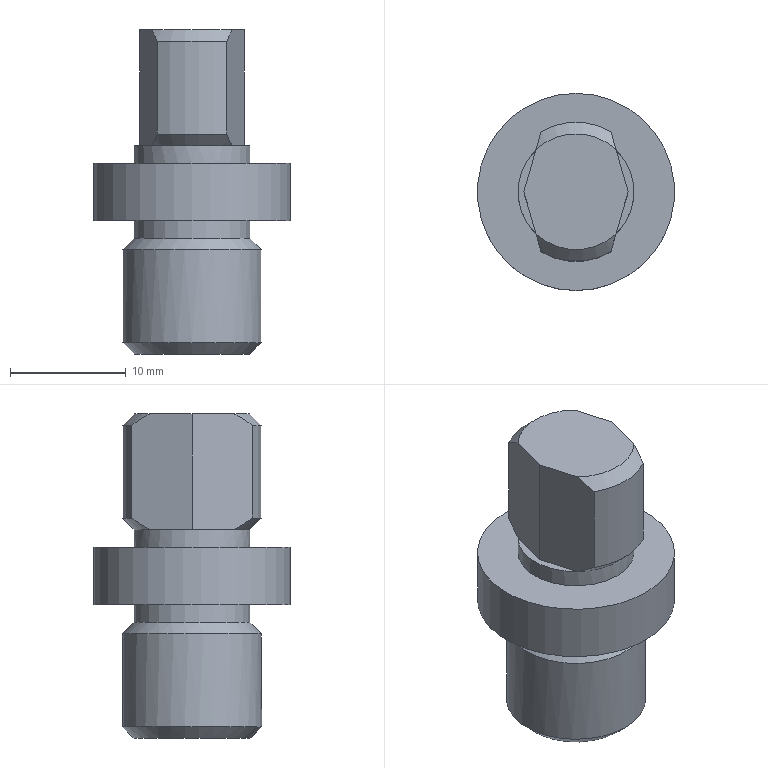Component | NX | B_LOCATING_PIN | 1 solid | 22 faces | volume 3297 mm3 | plane 10 | cylinder 6 | cone 6 | commonest cylinder face diameters 12 x3 10 x2 17 x1